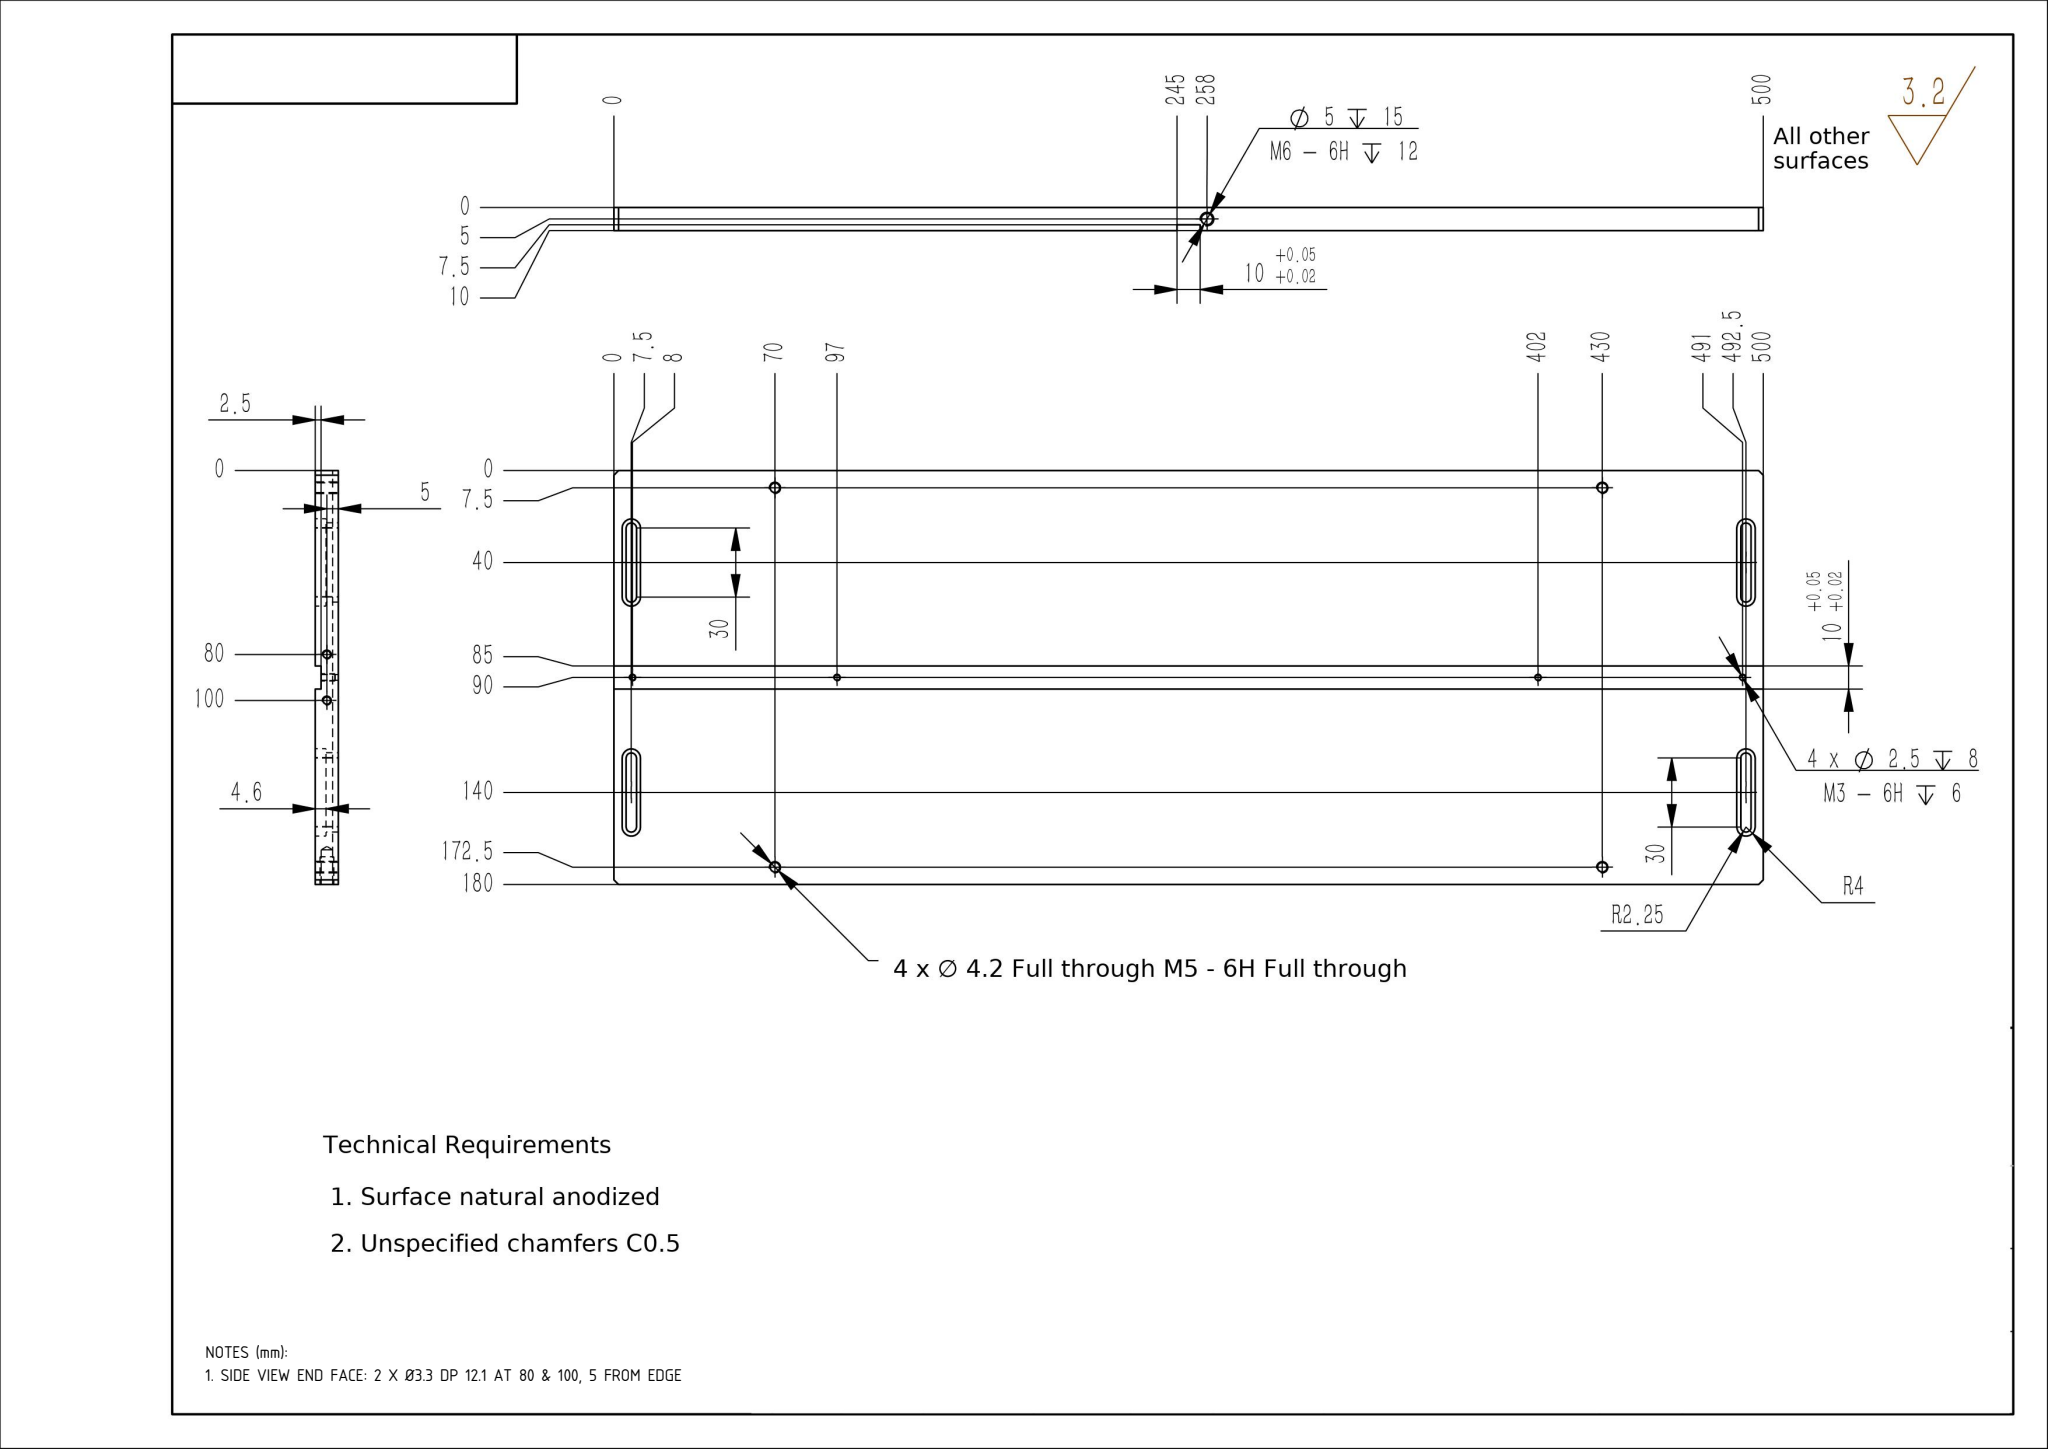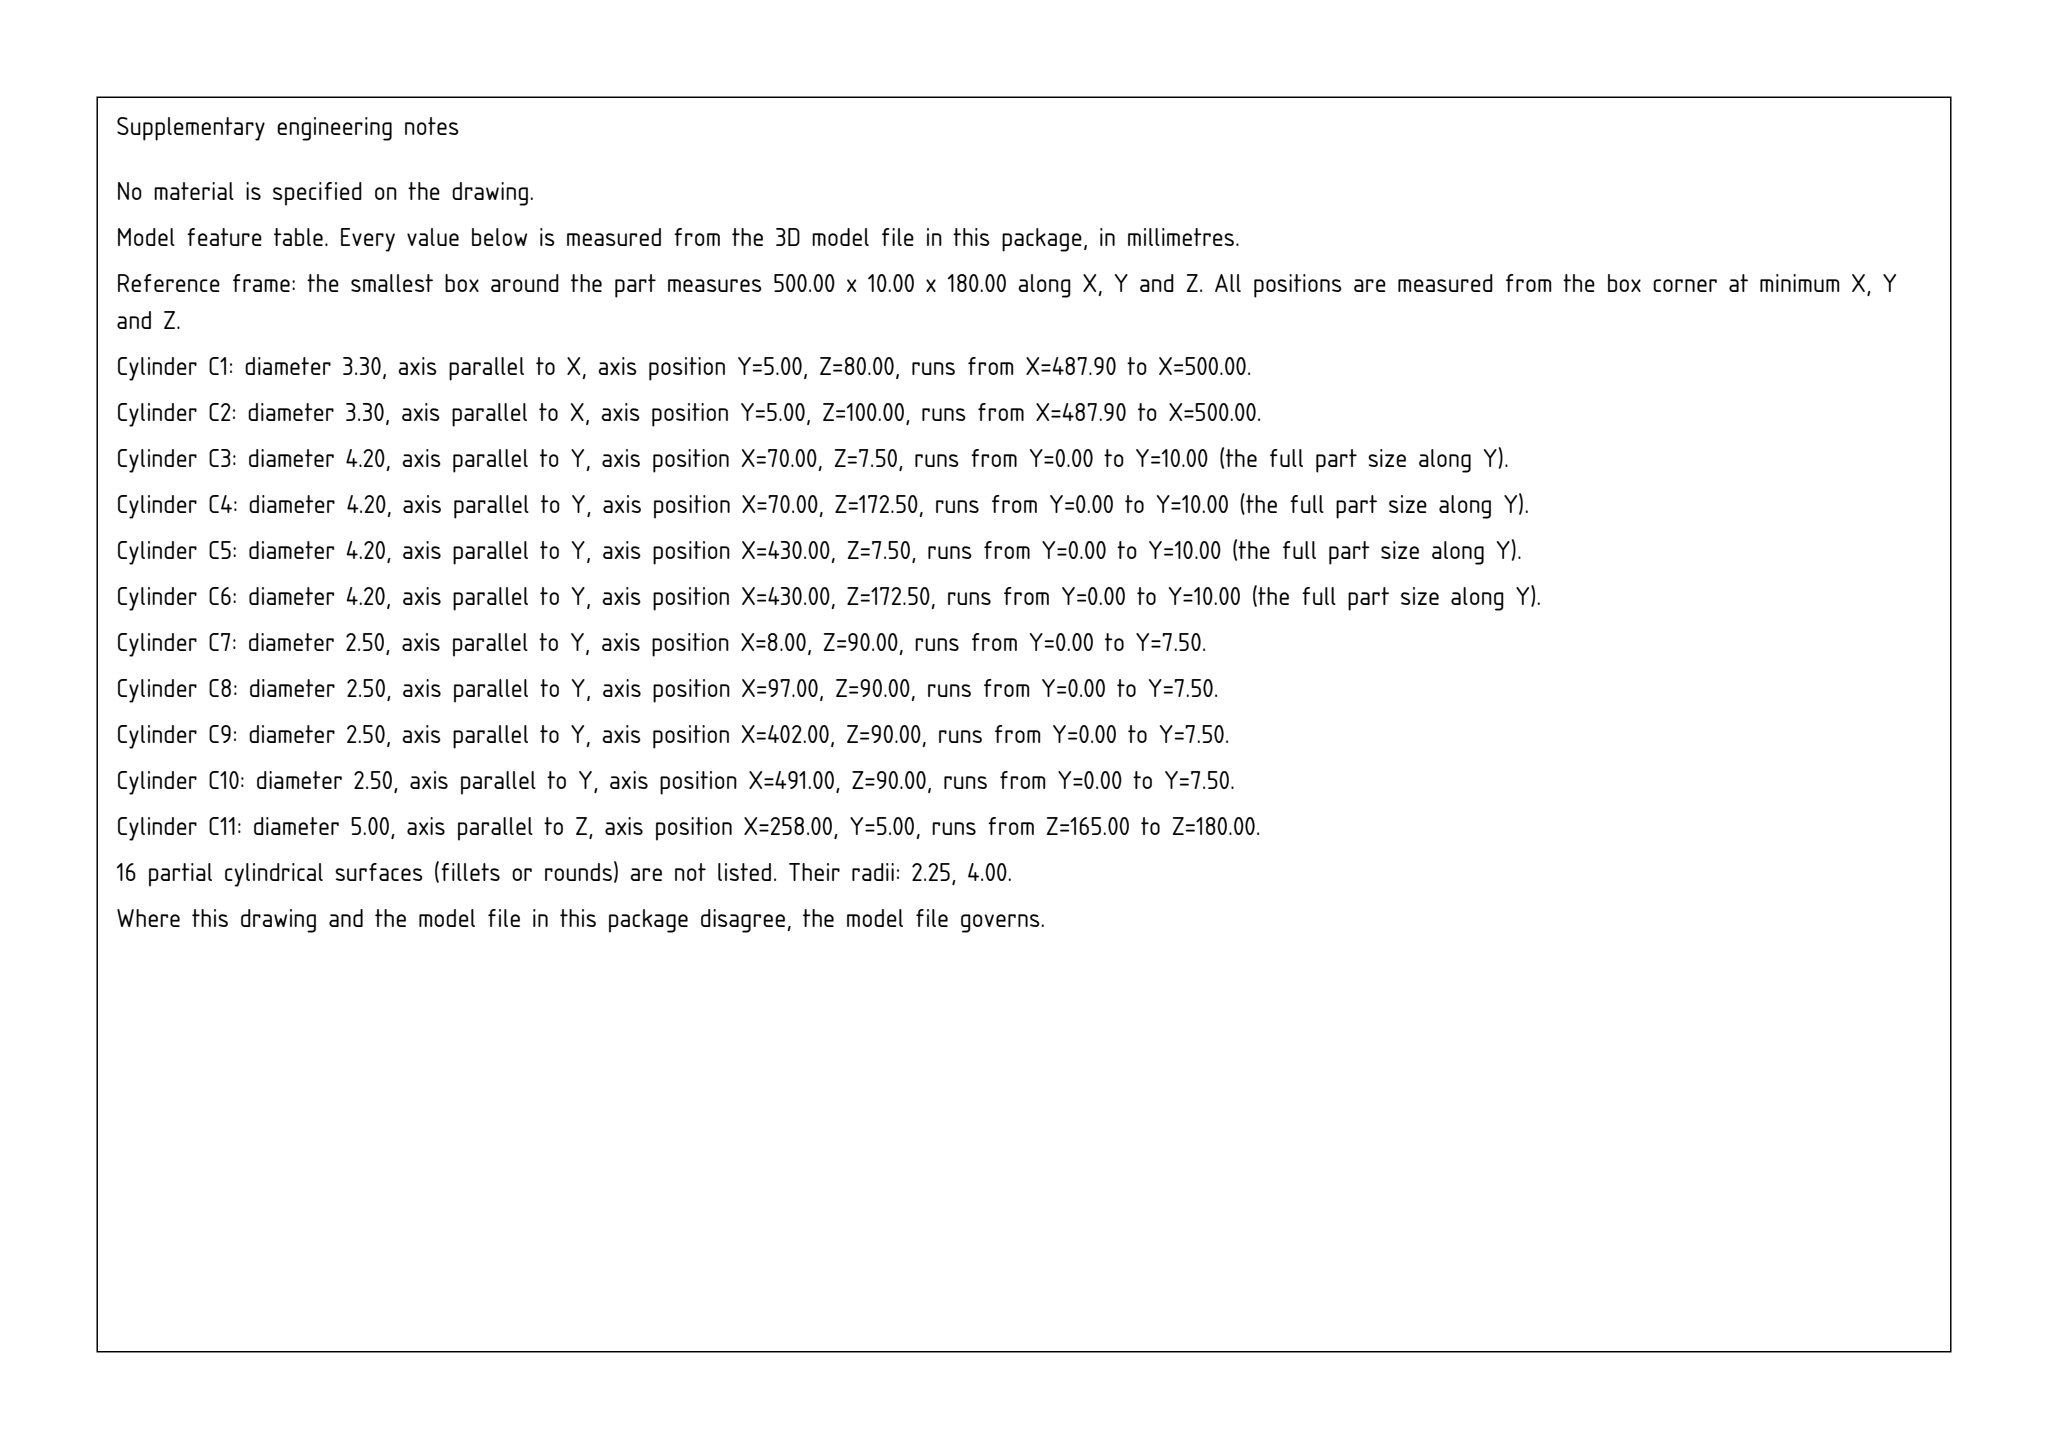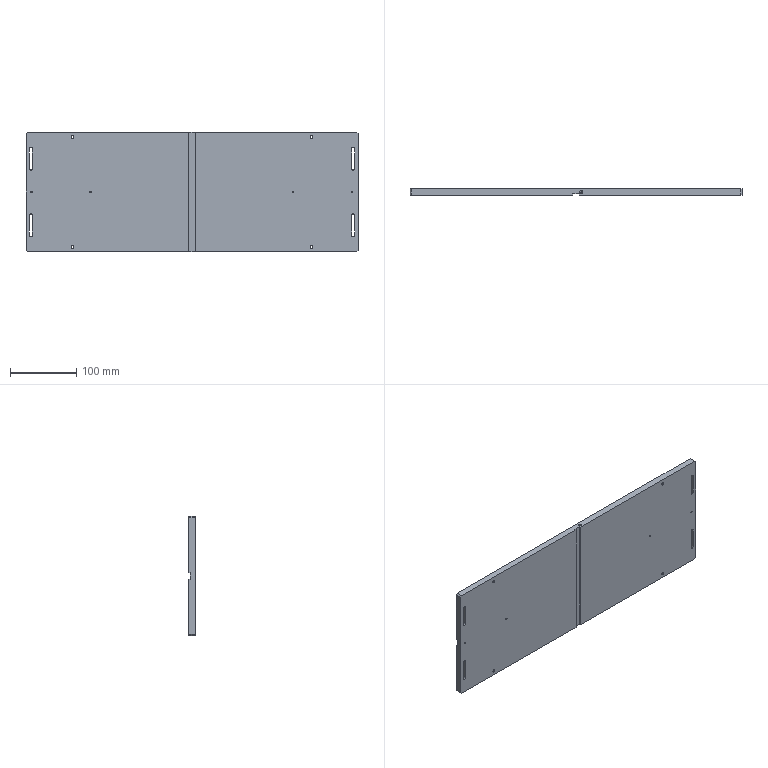Part | SolidWorks | mm | 1 solid | 90 faces | box 500 x 10 x 180 mm | volume 873101 mm3 | cylinder 46 | plane 38 | cone 6 | commonest cylinder face diameters 8 x12 4.5 x12 2.5 x8 4.2 x8 3.3 x4 5 x2
Drawing notes:
SIDE VIEW END FACE: 2 X Ø3.3 DP 12.1 AT 80 & 100, 5 FROM EDGE | from the solid: cylinders [3.3,"x",[null,5.0,80.0],12.1] and [3.3,"x",[null,5.0,100.0],12.1]; cones 118 deg ref dia 3.3 (drill point)
build123d program:
from build123d import *

# Parameters (mm, degrees)
SKETCH1_W             = 500
SKETCH1_H             = 180
BOSS_EXTRUDE1_DEPTH   = 10
SKETCH2_W             = 611.38
SKETCH2_H             = 10
CUT_EXTRUDE1_DEPTH    = 2.5
SKETCH3_W             = 10
SKETCH3_H             = 180
CUT_EXTRUDE2_DEPTH    = 2.5
CHAMFER1_SIZE         = 2
CUT_EXTRUDE3_DEPTH    = 10
M5_TAPPED_HOLE1_D     = 4.2
M4_TAPPED_HOLE1_D     = 3.3
M4_TAPPED_HOLE1_DEPTH = 12.1
M4_TAPPED_HOLE1_TIP   = 0.9914
M6_TAPPED_HOLE1_D     = 5
M6_TAPPED_HOLE1_DEPTH = 15
M6_TAPPED_HOLE1_TIP   = 1.502
M3_TAPPED_HOLE1_D     = 2.5
M3_TAPPED_HOLE1_DEPTH = 8
M3_TAPPED_HOLE1_TIP   = 0.7511
CUT_EXTRUDE4_DEPTH    = 4.6


with BuildPart() as part:
    # Sketch1 → Boss-Extrude1 (new body)
    with BuildSketch(Plane(origin=(0, 0, 0), x_dir=(1, 0, 0), z_dir=(0, 1, 0))):
        Rectangle(SKETCH1_W, SKETCH1_H)
    extrude(amount=BOSS_EXTRUDE1_DEPTH)

    # Sketch2 → Cut-Extrude1 (cut)
    with BuildSketch(Plane(origin=(0, 10, 0), x_dir=(1, 0, 0), z_dir=(0, 1, 0))):
        Rectangle(SKETCH2_W, SKETCH2_H)
    extrude(amount=-CUT_EXTRUDE1_DEPTH, mode=Mode.SUBTRACT)

    # Sketch3 → Cut-Extrude2 (cut)
    with BuildSketch(Plane.XZ):
        Rectangle(SKETCH3_W, SKETCH3_H)
    extrude(amount=-CUT_EXTRUDE2_DEPTH, mode=Mode.SUBTRACT)

    # Chamfer1
    chamfer1_edges = [part.edges().sort_by_distance(p)[0] for p in [
        (250, 5, 90),
        (-250, 5, 90),
        (-250, 5, -90),
        (250, 5, -90),
    ]]
    chamfer(chamfer1_edges, length=CHAMFER1_SIZE)

    # Sketch4 → Cut-Extrude3 (cut)
    with BuildSketch(Plane(origin=(0, 10, 0), x_dir=(1, 0, 0), z_dir=(0, 1, 0))):
        with BuildLine():
            Line((-240.25, 65), (-240.25, 35))
            ThreePointArc((-240.25, 35), (-242.5, 32.75), (-244.75, 35))
            Line((-244.75, 35), (-244.75, 65))
            ThreePointArc((-244.75, 65), (-242.5, 67.25), (-240.25, 65))
        make_face()
        with BuildLine():
            Line((240.25, 65), (240.25, 35))
            ThreePointArc((240.25, 35), (242.5, 32.75), (244.75, 35))
            Line((244.75, 35), (244.75, 65))
            ThreePointArc((244.75, 65), (242.5, 67.25), (240.25, 65))
        make_face()
        with BuildLine():
            Line((240.25, -65), (240.25, -35))
            ThreePointArc((240.25, -35), (242.5, -32.75), (244.75, -35))
            Line((244.75, -35), (244.75, -65))
            ThreePointArc((244.75, -65), (242.5, -67.25), (240.25, -65))
        make_face()
        with BuildLine():
            Line((-240.25, -65), (-240.25, -35))
            ThreePointArc((-240.25, -35), (-242.5, -32.75), (-244.75, -35))
            Line((-244.75, -35), (-244.75, -65))
            ThreePointArc((-244.75, -65), (-242.5, -67.25), (-240.25, -65))
        make_face()
    extrude(amount=-CUT_EXTRUDE3_DEPTH, mode=Mode.SUBTRACT)

    # M5 Tapped Hole1 (through all)
    with Locations(Plane(origin=(0, 10, 0), x_dir=(1, 0, 0), z_dir=(0, 1, 0))):
        with Locations((-180, -82.5), (-180, 82.5), (180, -82.5), (180, 82.5)):
            Hole(M5_TAPPED_HOLE1_D / 2)

    # M4 Tapped Hole1
    with Locations(Plane(origin=(250, 0, 0), x_dir=(0, 0, -1), z_dir=(1, 0, 0))):
        with Locations((-10, 5), (10, 5)):
            Hole(M4_TAPPED_HOLE1_D / 2, depth=M4_TAPPED_HOLE1_DEPTH)
            with Locations((0, 0, -(M4_TAPPED_HOLE1_DEPTH + M4_TAPPED_HOLE1_TIP / 2))):  # 118° drill point
                Cone(0, M4_TAPPED_HOLE1_D / 2, M4_TAPPED_HOLE1_TIP, mode=Mode.SUBTRACT)

    # M6 Tapped Hole1
    with Locations(Plane.XY.offset(90)):
        with Locations((8, 5)):
            Hole(M6_TAPPED_HOLE1_D / 2, depth=M6_TAPPED_HOLE1_DEPTH)
            with Locations((0, 0, -(M6_TAPPED_HOLE1_DEPTH + M6_TAPPED_HOLE1_TIP / 2))):  # 118° drill point
                Cone(0, M6_TAPPED_HOLE1_D / 2, M6_TAPPED_HOLE1_TIP, mode=Mode.SUBTRACT)

    # M3 Tapped Hole1
    with Locations(Plane(origin=(0, 7.5, 0), x_dir=(1, 0, 0), z_dir=(0, 1, 0))):
        with Locations((241, 0), (152, 0), (-153, 0), (-242, 0)):
            Hole(M3_TAPPED_HOLE1_D / 2, depth=M3_TAPPED_HOLE1_DEPTH)
            with Locations((0, 0, -(M3_TAPPED_HOLE1_DEPTH + M3_TAPPED_HOLE1_TIP / 2))):  # 118° drill point
                Cone(0, M3_TAPPED_HOLE1_D / 2, M3_TAPPED_HOLE1_TIP, mode=Mode.SUBTRACT)

    # Sketch15 → Cut-Extrude4 (cut)
    with BuildSketch(Plane(origin=(0, 10, 0), x_dir=(1, 0, 0), z_dir=(0, 1, 0))):
        with BuildLine():
            Line((-238.5, 65), (-238.5, 35))
            ThreePointArc((-238.5, 35), (-242.5, 31), (-246.5, 35))
            Line((-246.5, 35), (-246.5, 65))
            ThreePointArc((-246.5, 65), (-242.5, 69), (-238.5, 65))
        make_face()
        with BuildLine():
            Line((-238.5, -35), (-238.5, -65))
            ThreePointArc((-238.5, -65), (-242.5, -69), (-246.5, -65))
            Line((-246.5, -65), (-246.5, -35))
            ThreePointArc((-246.5, -35), (-242.5, -31), (-238.5, -35))
        make_face()
        with BuildLine():
            Line((246.5, 65), (246.5, 35))
            ThreePointArc((246.5, 35), (242.5, 31), (238.5, 35))
            Line((238.5, 35), (238.5, 65))
            ThreePointArc((238.5, 65), (242.5, 69), (246.5, 65))
        make_face()
        with BuildLine():
            Line((246.5, -35), (246.5, -65))
            ThreePointArc((246.5, -65), (242.5, -69), (238.5, -65))
            Line((238.5, -65), (238.5, -35))
            ThreePointArc((238.5, -35), (242.5, -31), (246.5, -35))
        make_face()
    extrude(amount=-CUT_EXTRUDE4_DEPTH, mode=Mode.SUBTRACT)


solid = part.part